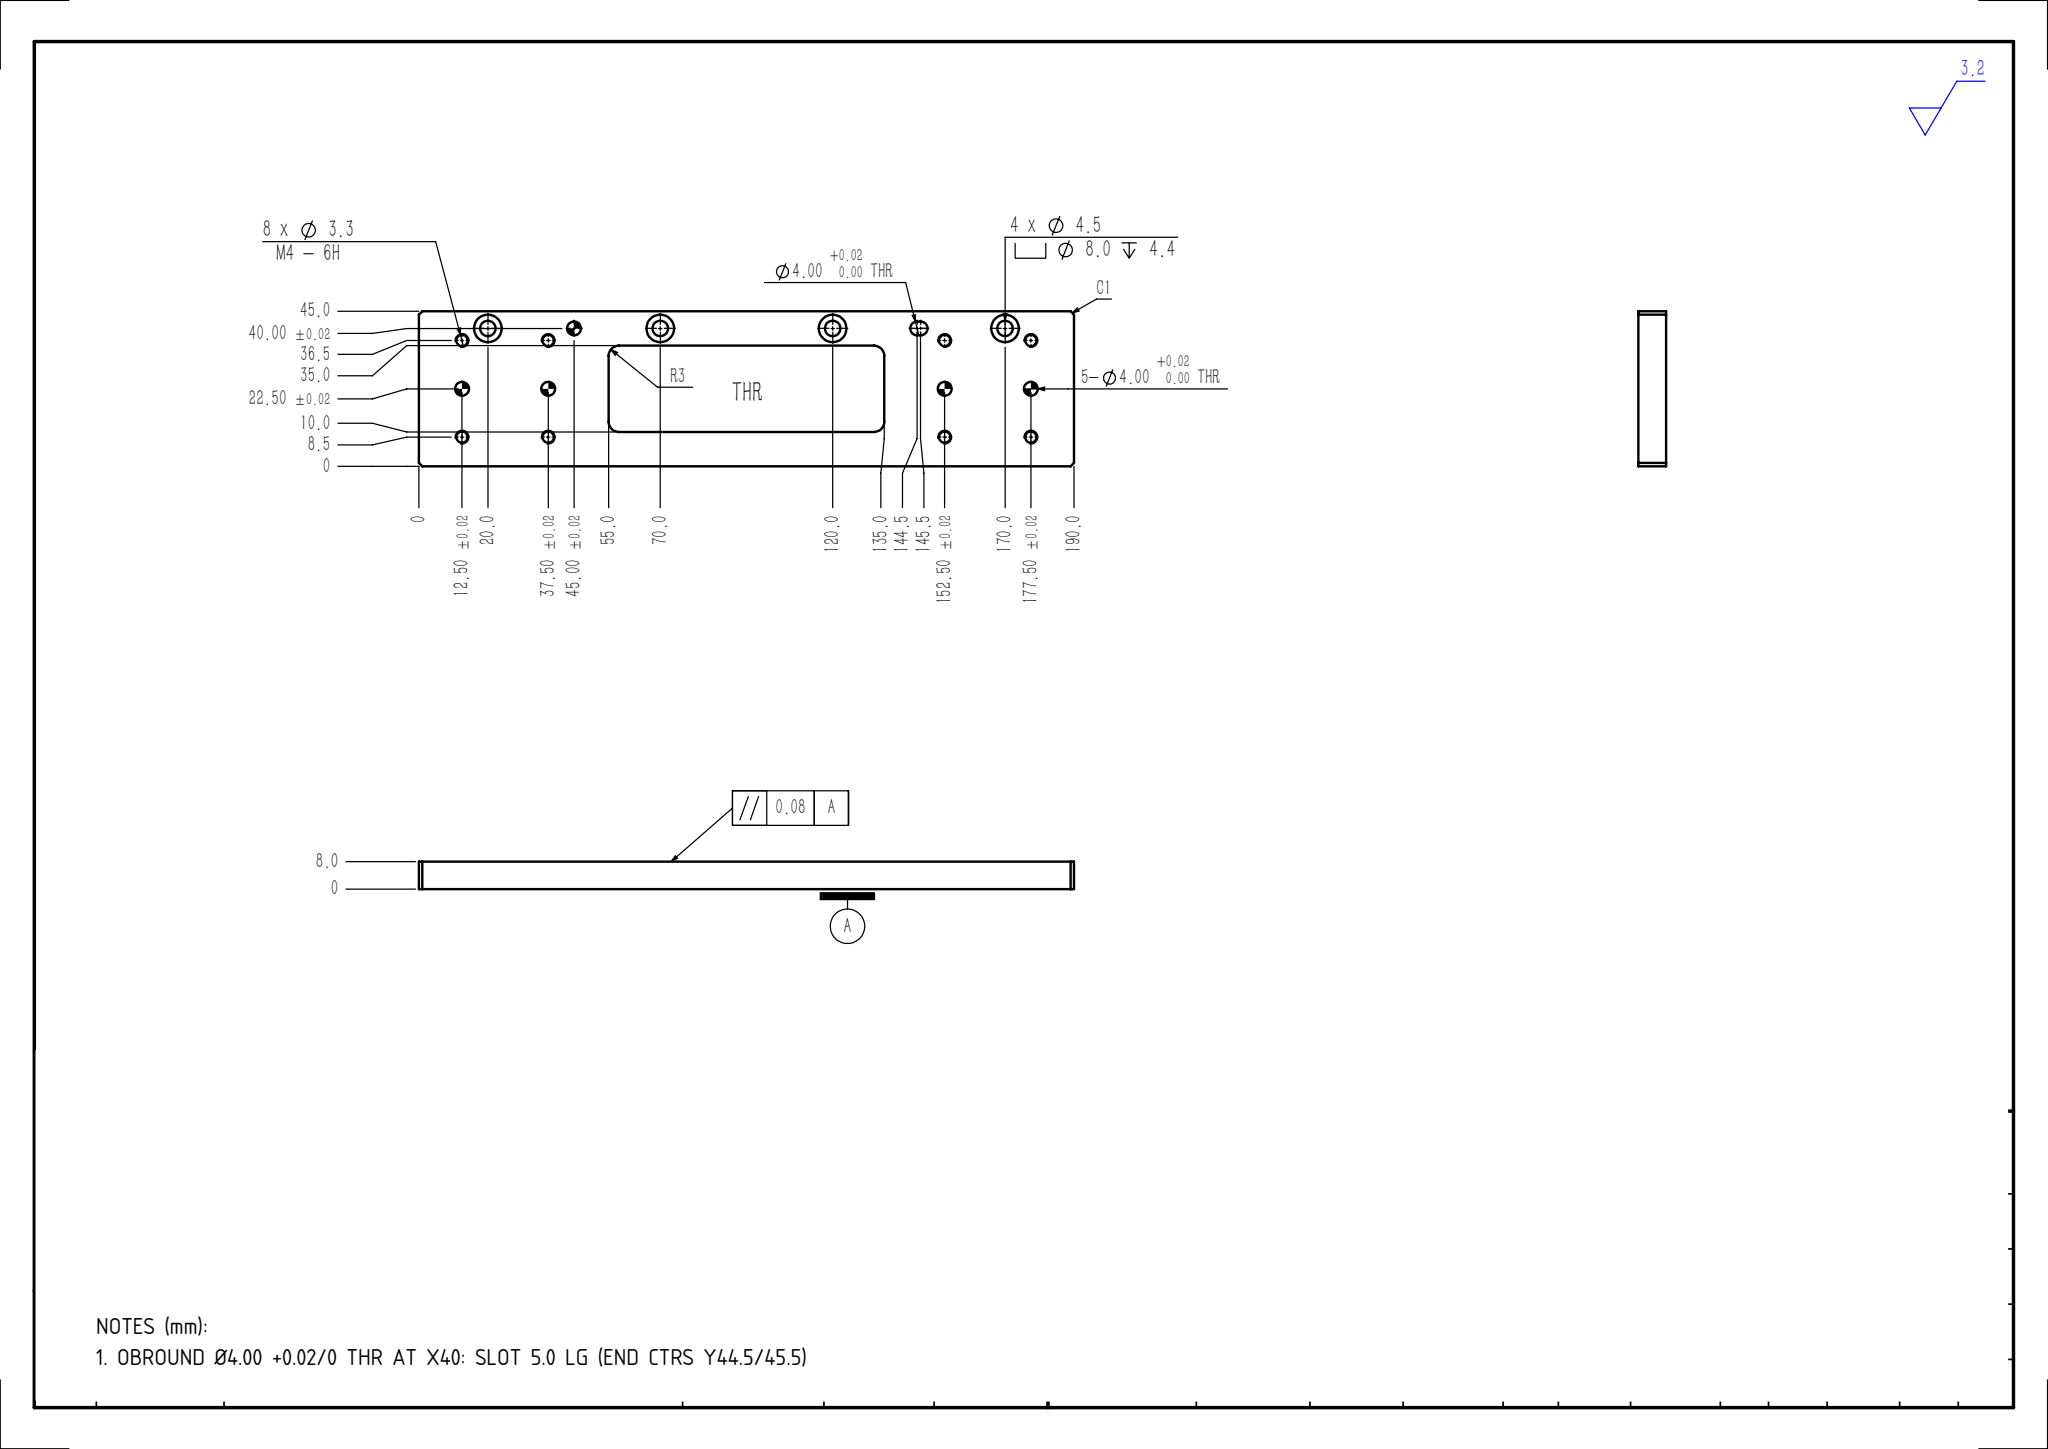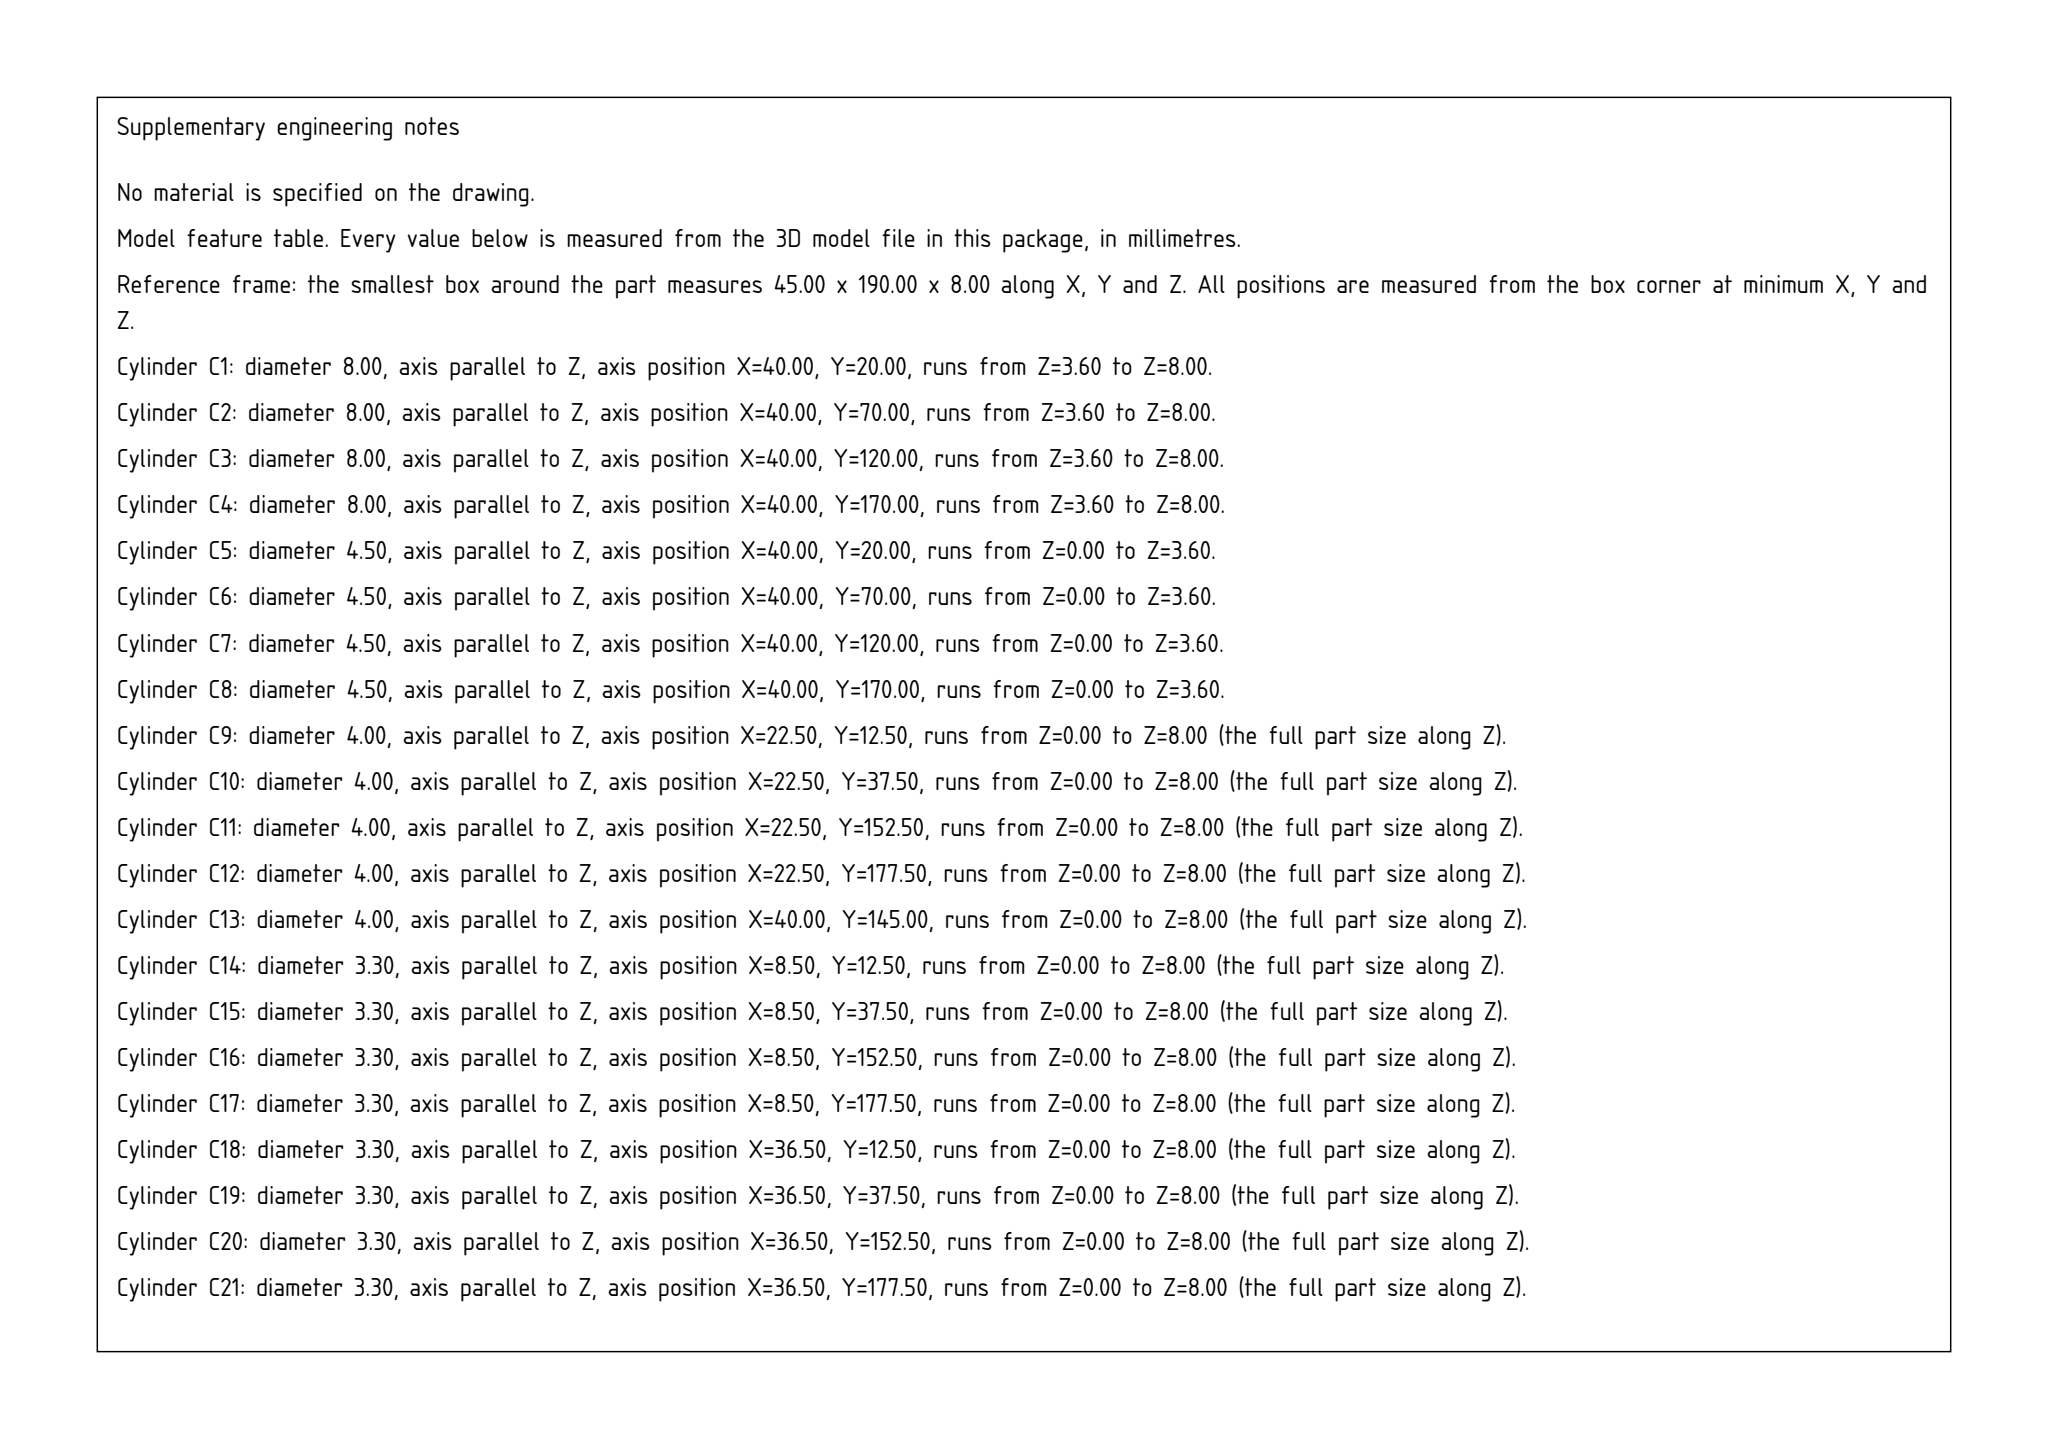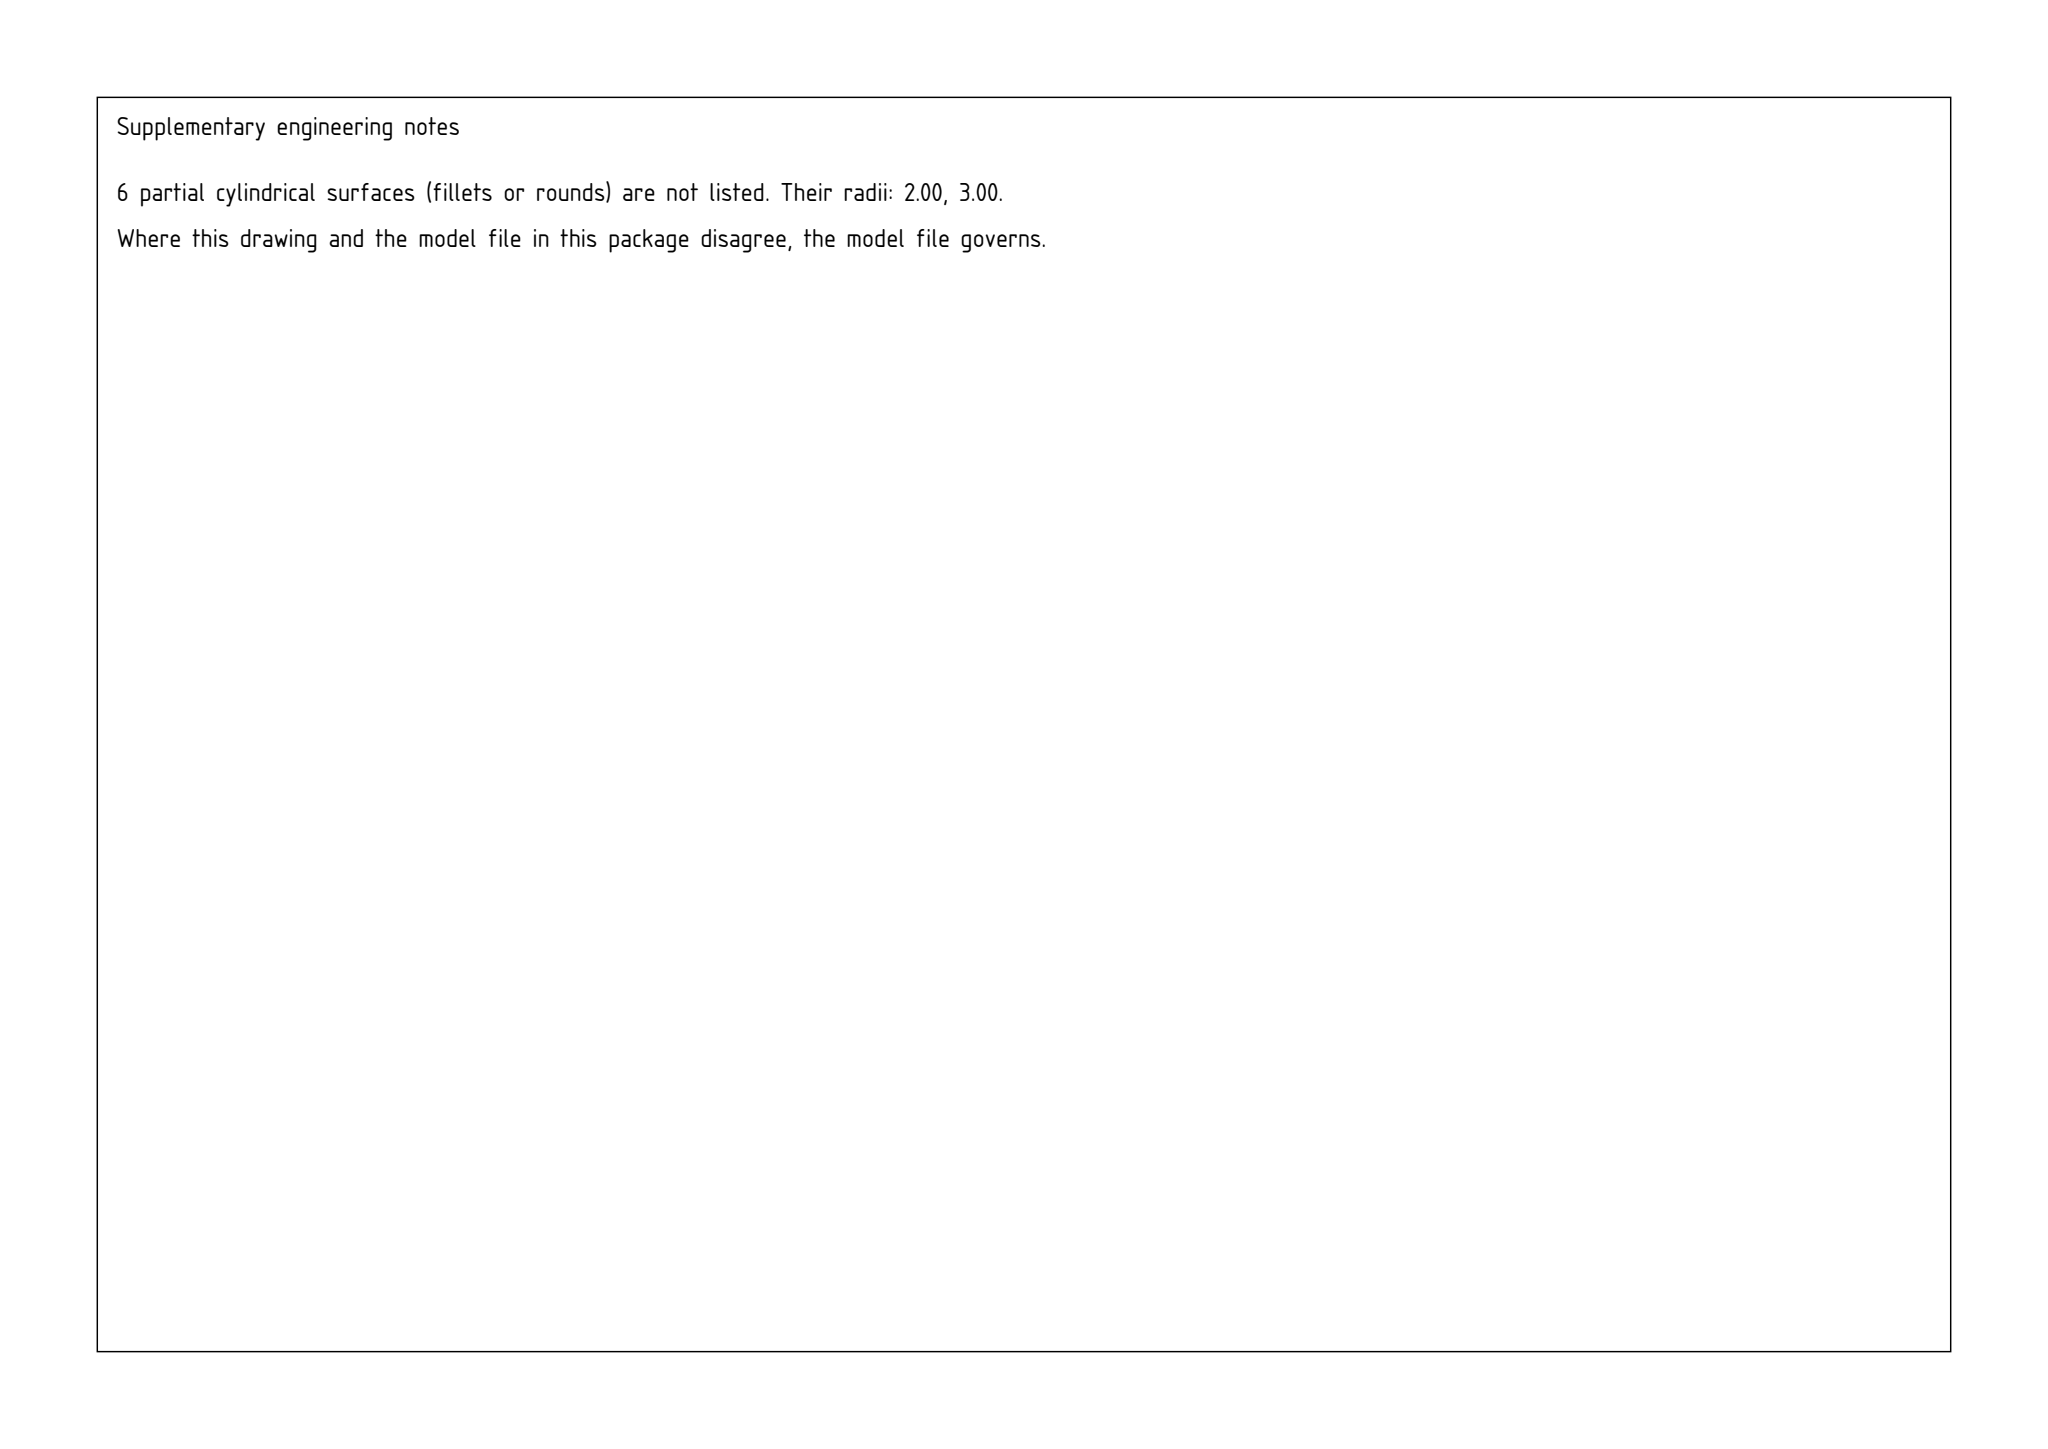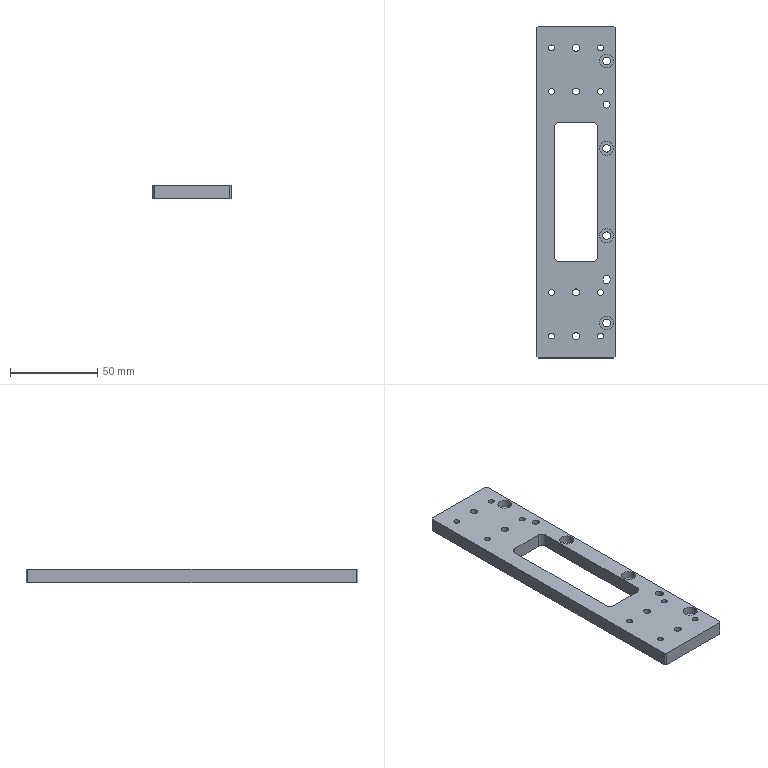Part | SolidWorks | mm | 1 solid | 68 faces | box 45 x 190 x 8 mm | volume 50150 mm3 | cylinder 48 | plane 20 | commonest cylinder face diameters 3.3 x16 4 x12 8 x8 4.5 x8 6 x4
Drawing notes:
OBROUND Ø4.00 +0.02/0 THR AT X40: SLOT 5.0 LG (END CTRS Y44.5/45.5) | from the solid: Two Ø4.0 z-cylinders at (x=40,y=44.5) and (x=40,y=45.5), len 8.0 thru; 1.0 c-c + Ø4 = 5.0 overall
build123d program:
from build123d import *

# Parameters (mm, degrees)
SKETCH1_W                                       = 45
SKETCH1_H                                       = 190
BOSS_EXTRUDE1_DEPTH                             = 8
SKETCH2_W                                       = 25
SKETCH2_H                                       = 80
CUT_EXTRUDE1_DEPTH                              = 98.955
FILLET1_R                                       = 3
M4_HEX_SOCKET_HEAD_CAP_SCREW_CBORE2_D           = 4.5
M4_HEX_SOCKET_HEAD_CAP_SCREW_CBORE2_CBORE_D     = 8
M4_HEX_SOCKET_HEAD_CAP_SCREW_CBORE2_CBORE_DEPTH = 4.4
SKETCH6_R                                       = 2
CUT_EXTRUDE2_DEPTH                              = 98.955
M4_TAPPED_HOLE1_D                               = 3.3
SIZE_MM_DOWEL_PIN_HOLE1_D                       = 4
CHAMFER1_SIZE                                   = 1


with BuildPart() as part:
    # Sketch1 → Boss-Extrude1 (new body)
    with BuildSketch(Plane.XY):
        Rectangle(SKETCH1_W, SKETCH1_H)
    extrude(amount=BOSS_EXTRUDE1_DEPTH)

    # Sketch2 → Cut-Extrude1 (cut, through all)
    with BuildSketch(Plane.XY.offset(8)):
        Rectangle(SKETCH2_W, SKETCH2_H)
    extrude(amount=-CUT_EXTRUDE1_DEPTH, mode=Mode.SUBTRACT)

    # Fillet1
    fillet1_edges = [part.edges().sort_by_distance(p)[0] for p in [
        (12.5, 40, 4),
        (12.5, -40, 4),
        (-12.5, -40, 4),
        (-12.5, 40, 4),
    ]]
    fillet(fillet1_edges, radius=FILLET1_R)

    # M4 Hex Socket Head Cap Screw CBORE2 (through all)
    with Locations(Plane.XY.offset(8)):
        with Locations((17.5, 75), (17.5, 25), (17.5, -25), (17.5, -75)):
            CounterBoreHole(M4_HEX_SOCKET_HEAD_CAP_SCREW_CBORE2_D / 2, M4_HEX_SOCKET_HEAD_CAP_SCREW_CBORE2_CBORE_D / 2, M4_HEX_SOCKET_HEAD_CAP_SCREW_CBORE2_CBORE_DEPTH)

    # Sketch6 → Cut-Extrude2 (cut, through all)
    with BuildSketch(Plane.XY.offset(8)):
        with Locations((17.5, 50)):
            Circle(SKETCH6_R)
        with BuildLine():
            Line((19.5, -49.5), (19.5, -50.5))
            ThreePointArc((19.5, -50.5), (17.5, -52.5), (15.5, -50.5))
            Line((15.5, -50.5), (15.5, -49.5))
            ThreePointArc((15.5, -49.5), (17.5, -47.5), (19.5, -49.5))
        make_face()
    extrude(amount=-CUT_EXTRUDE2_DEPTH, mode=Mode.SUBTRACT)

    # M4 Tapped Hole1 (through all)
    with Locations(Plane.XY.offset(8)):
        with Locations((14, -57.5), (14, -82.5), (-14, -57.5), (-14, -82.5)):
            m4_tapped_hole1 = Hole(M4_TAPPED_HOLE1_D / 2)

    # Size mm Dowel Pin Hole1 (through all)
    with Locations(Plane.XY.offset(8)):
        with Locations((0, -82.5), (0, -57.5)):
            size_mm_dowel_pin_hole1 = Hole(SIZE_MM_DOWEL_PIN_HOLE1_D / 2)

    # Mirror1: M4 Tapped Hole1, Size mm Dowel Pin Hole1 across plane
    add(m4_tapped_hole1.mirror(Plane.ZX), mode=Mode.SUBTRACT)
    add(size_mm_dowel_pin_hole1.mirror(Plane.ZX), mode=Mode.SUBTRACT)

    # Chamfer1
    chamfer1_edges = [part.edges().sort_by_distance(p)[0] for p in [
        (22.5, -95, 4),
        (-22.5, -95, 4),
        (-22.5, 95, 4),
        (22.5, 95, 4),
    ]]
    chamfer(chamfer1_edges, length=CHAMFER1_SIZE)


solid = part.part